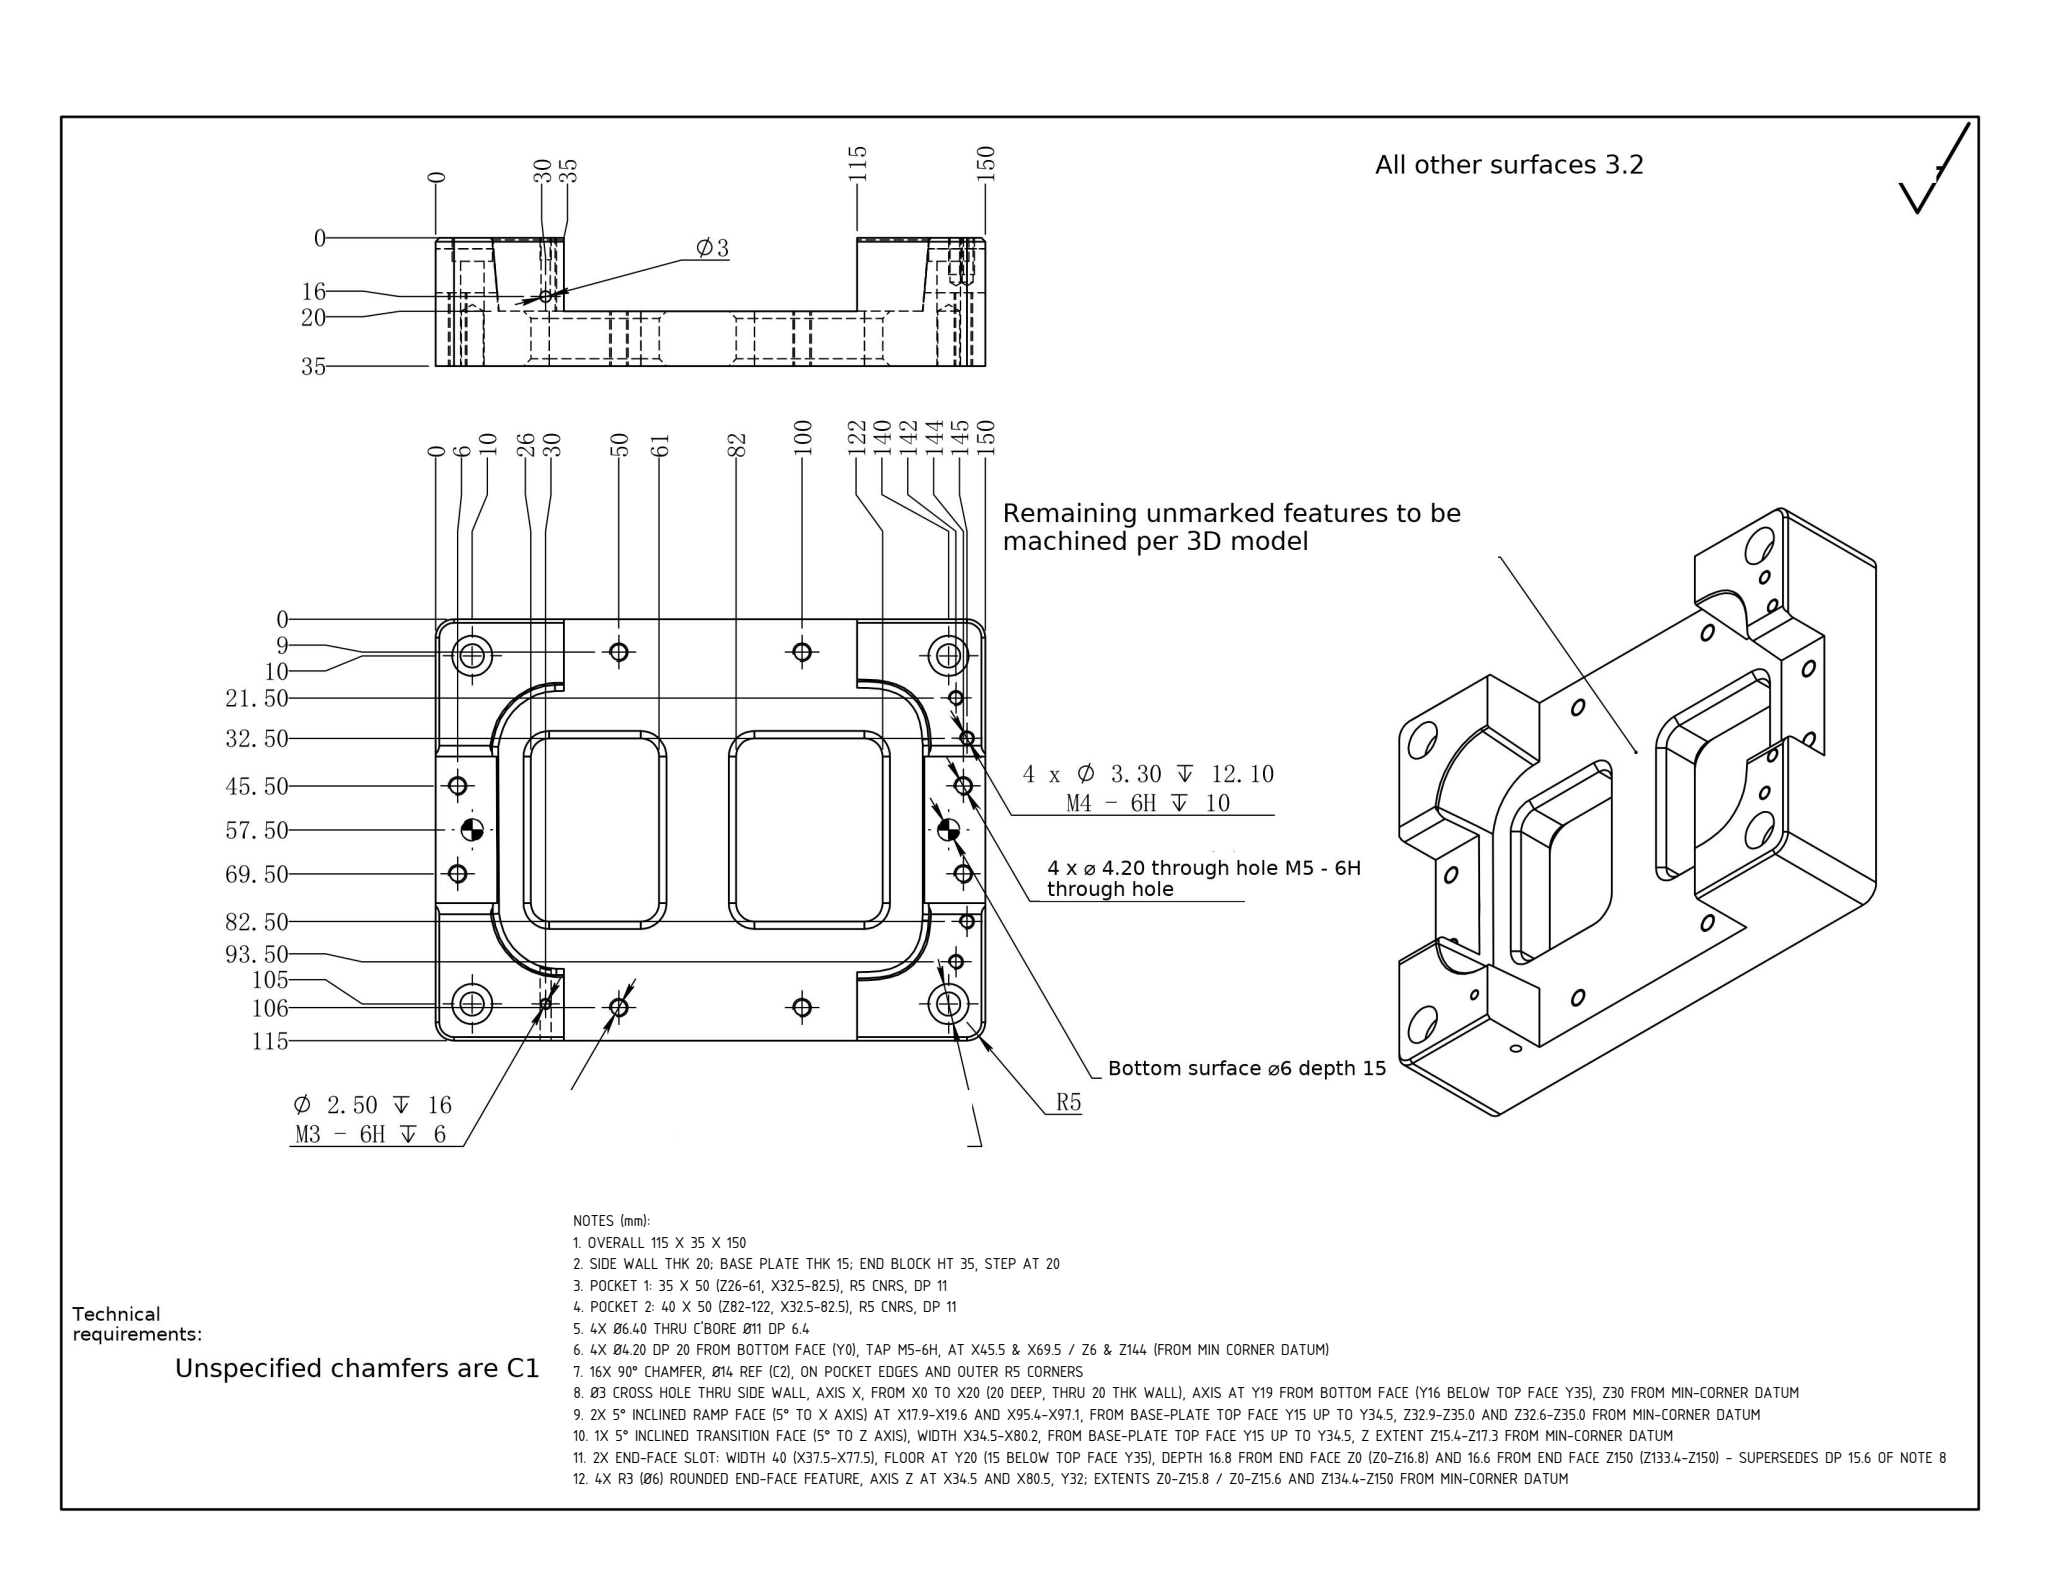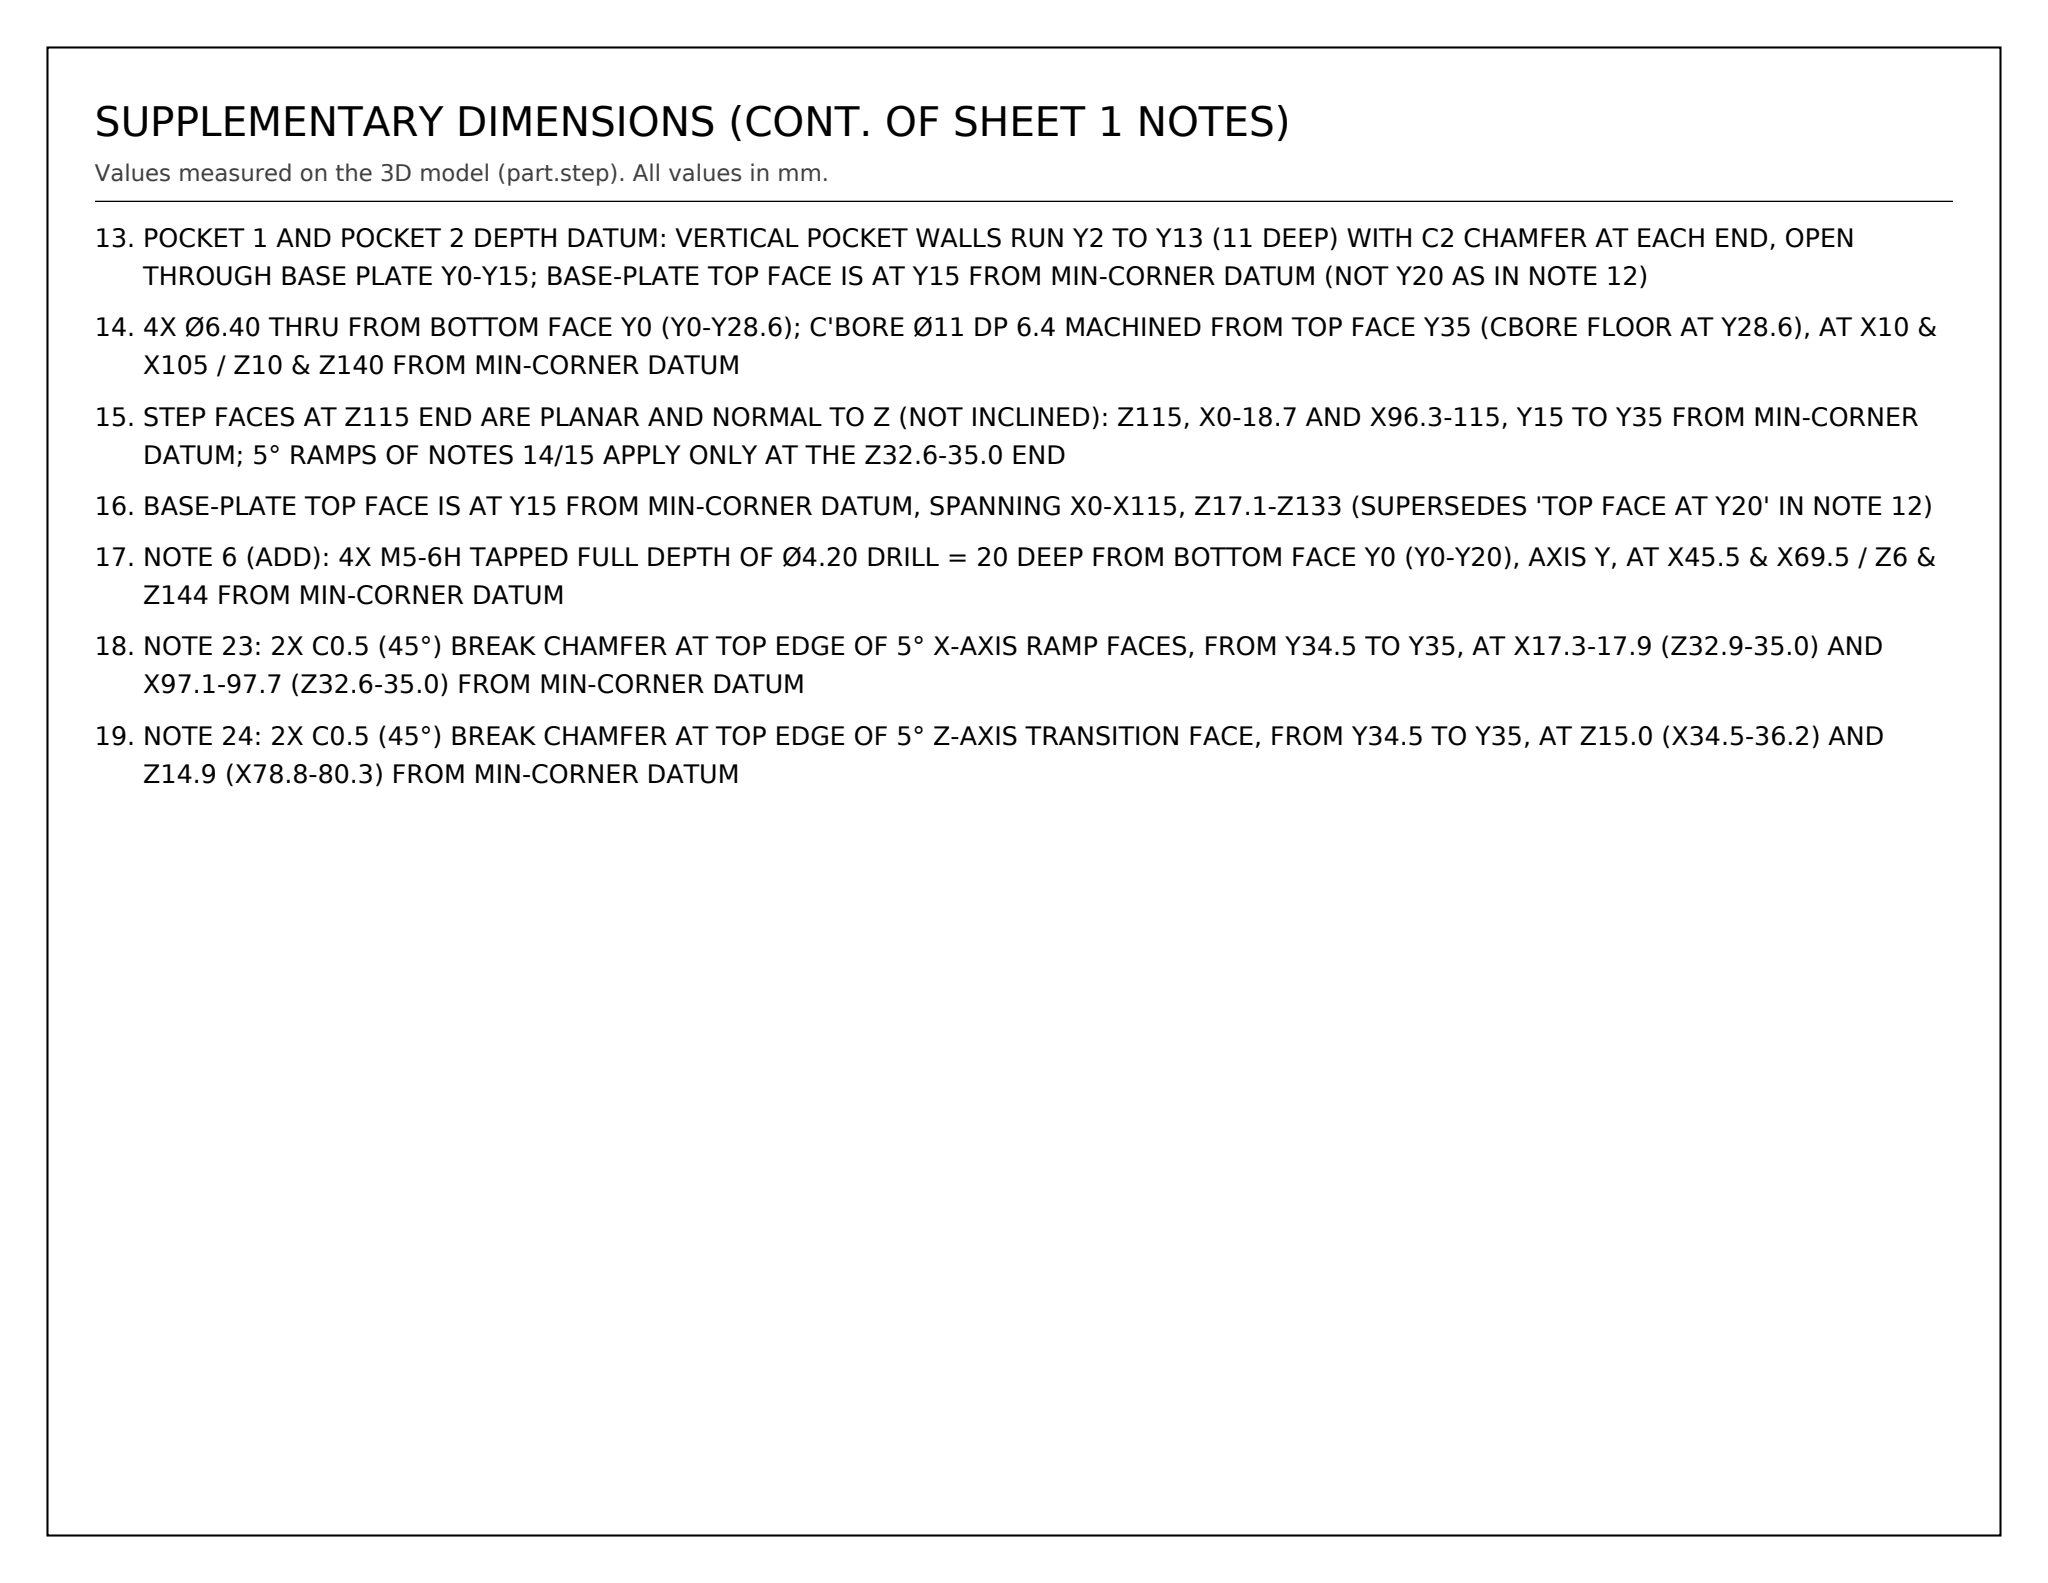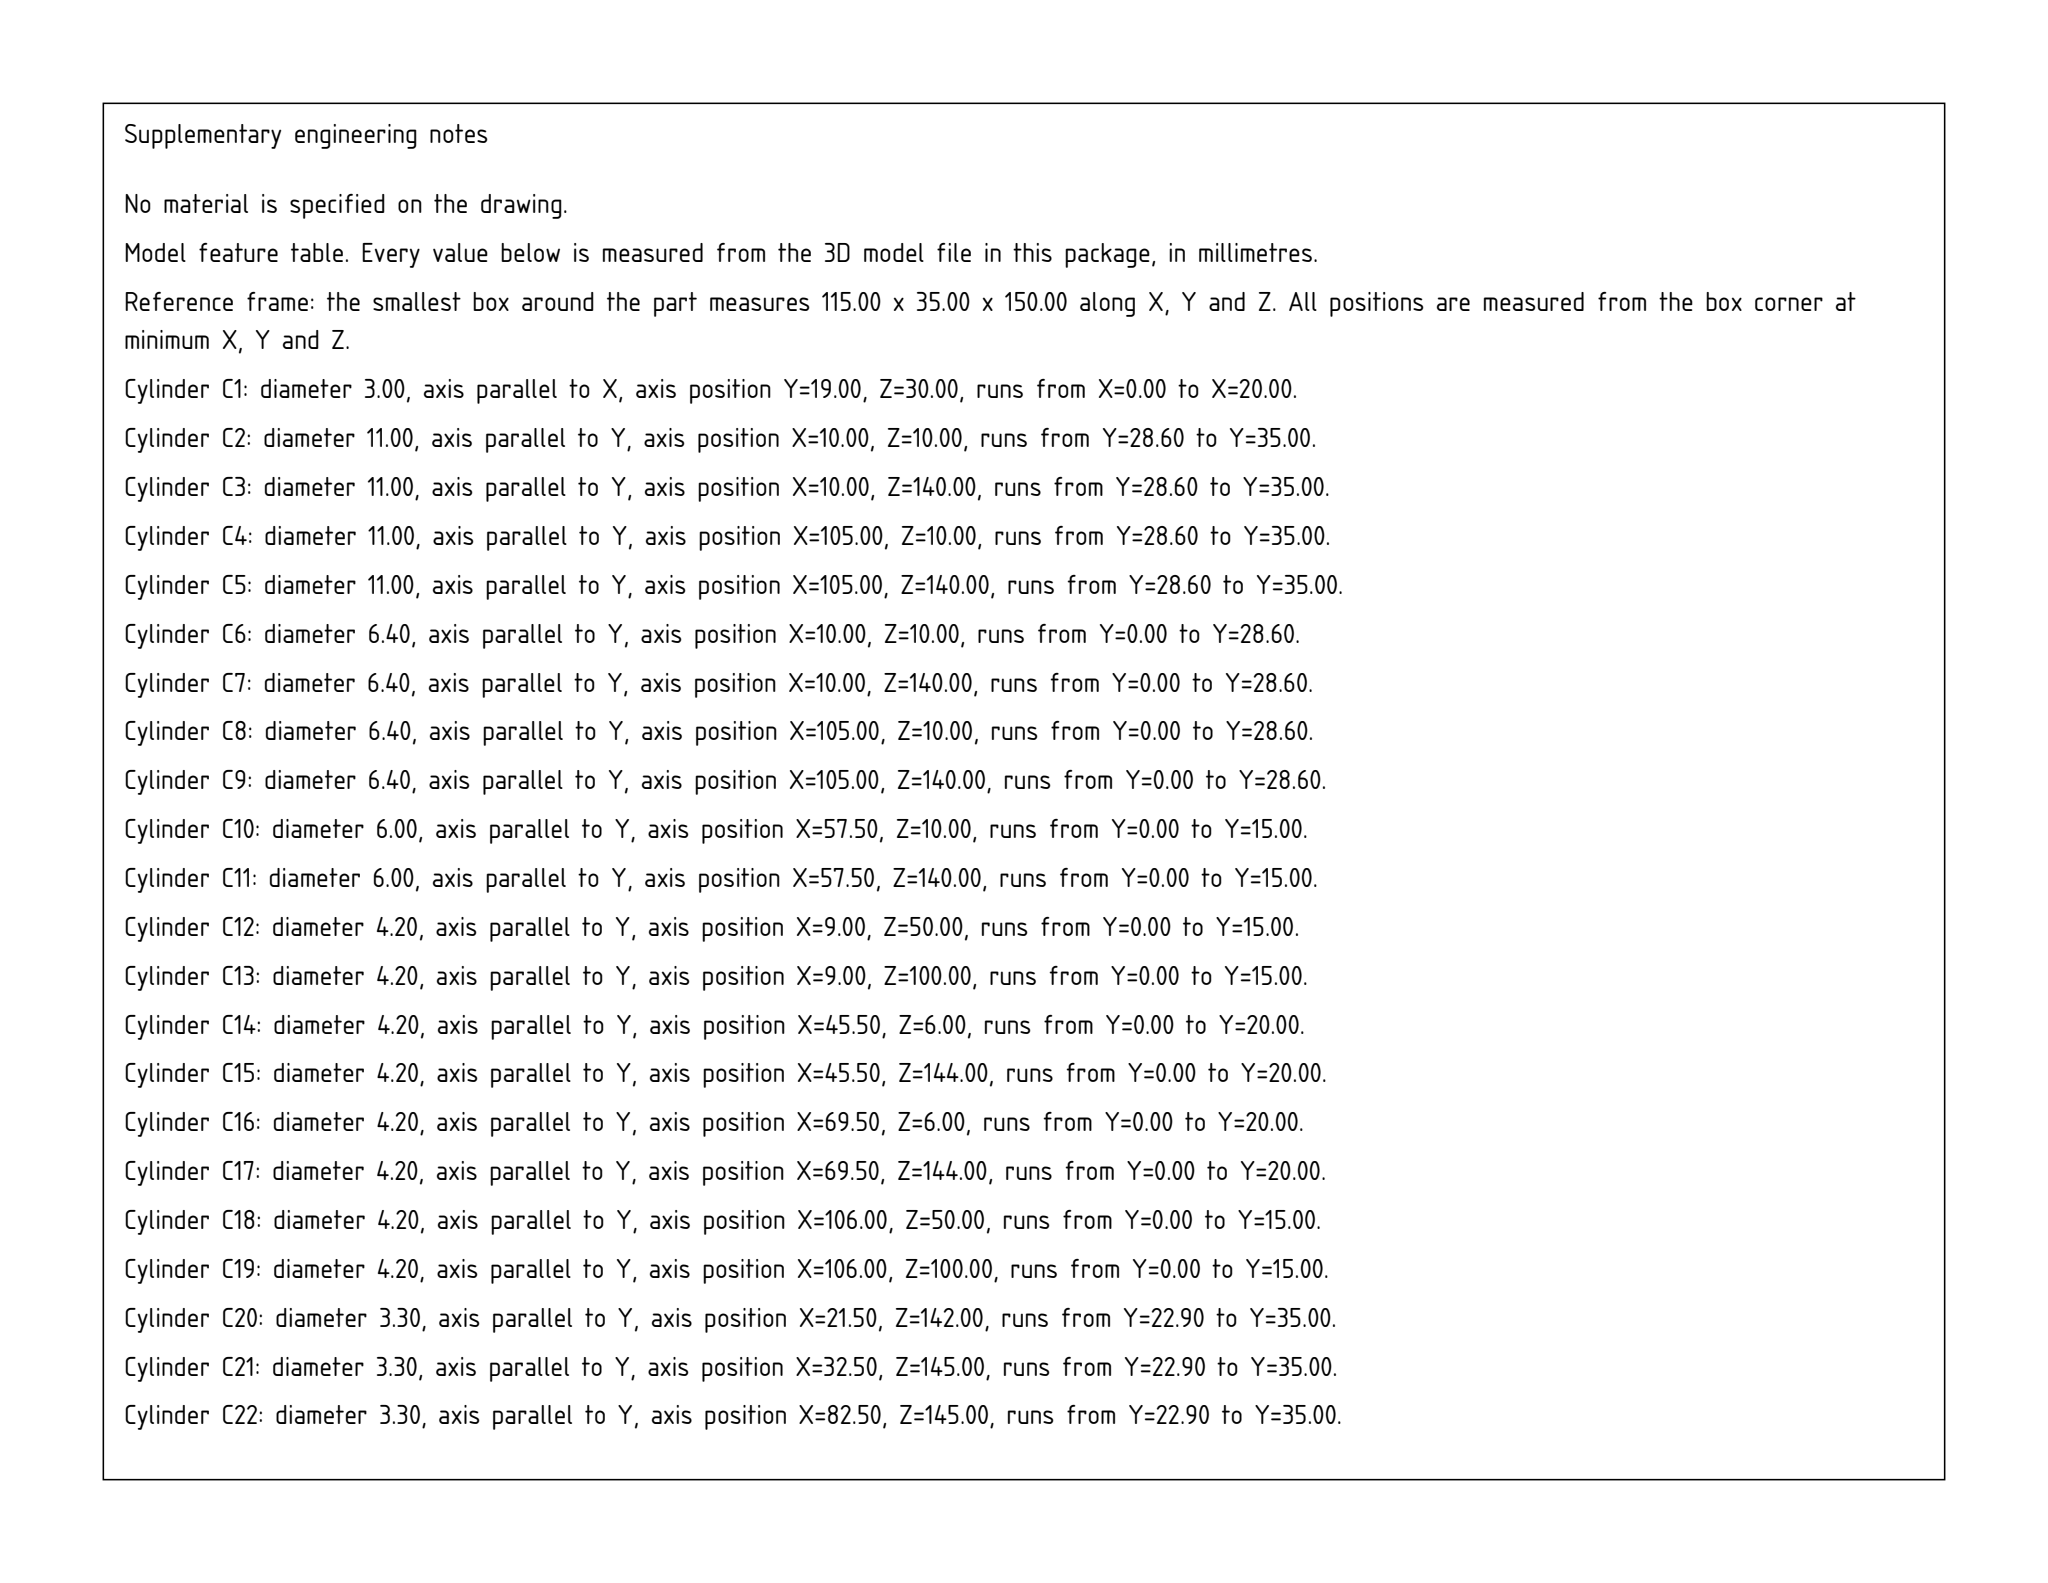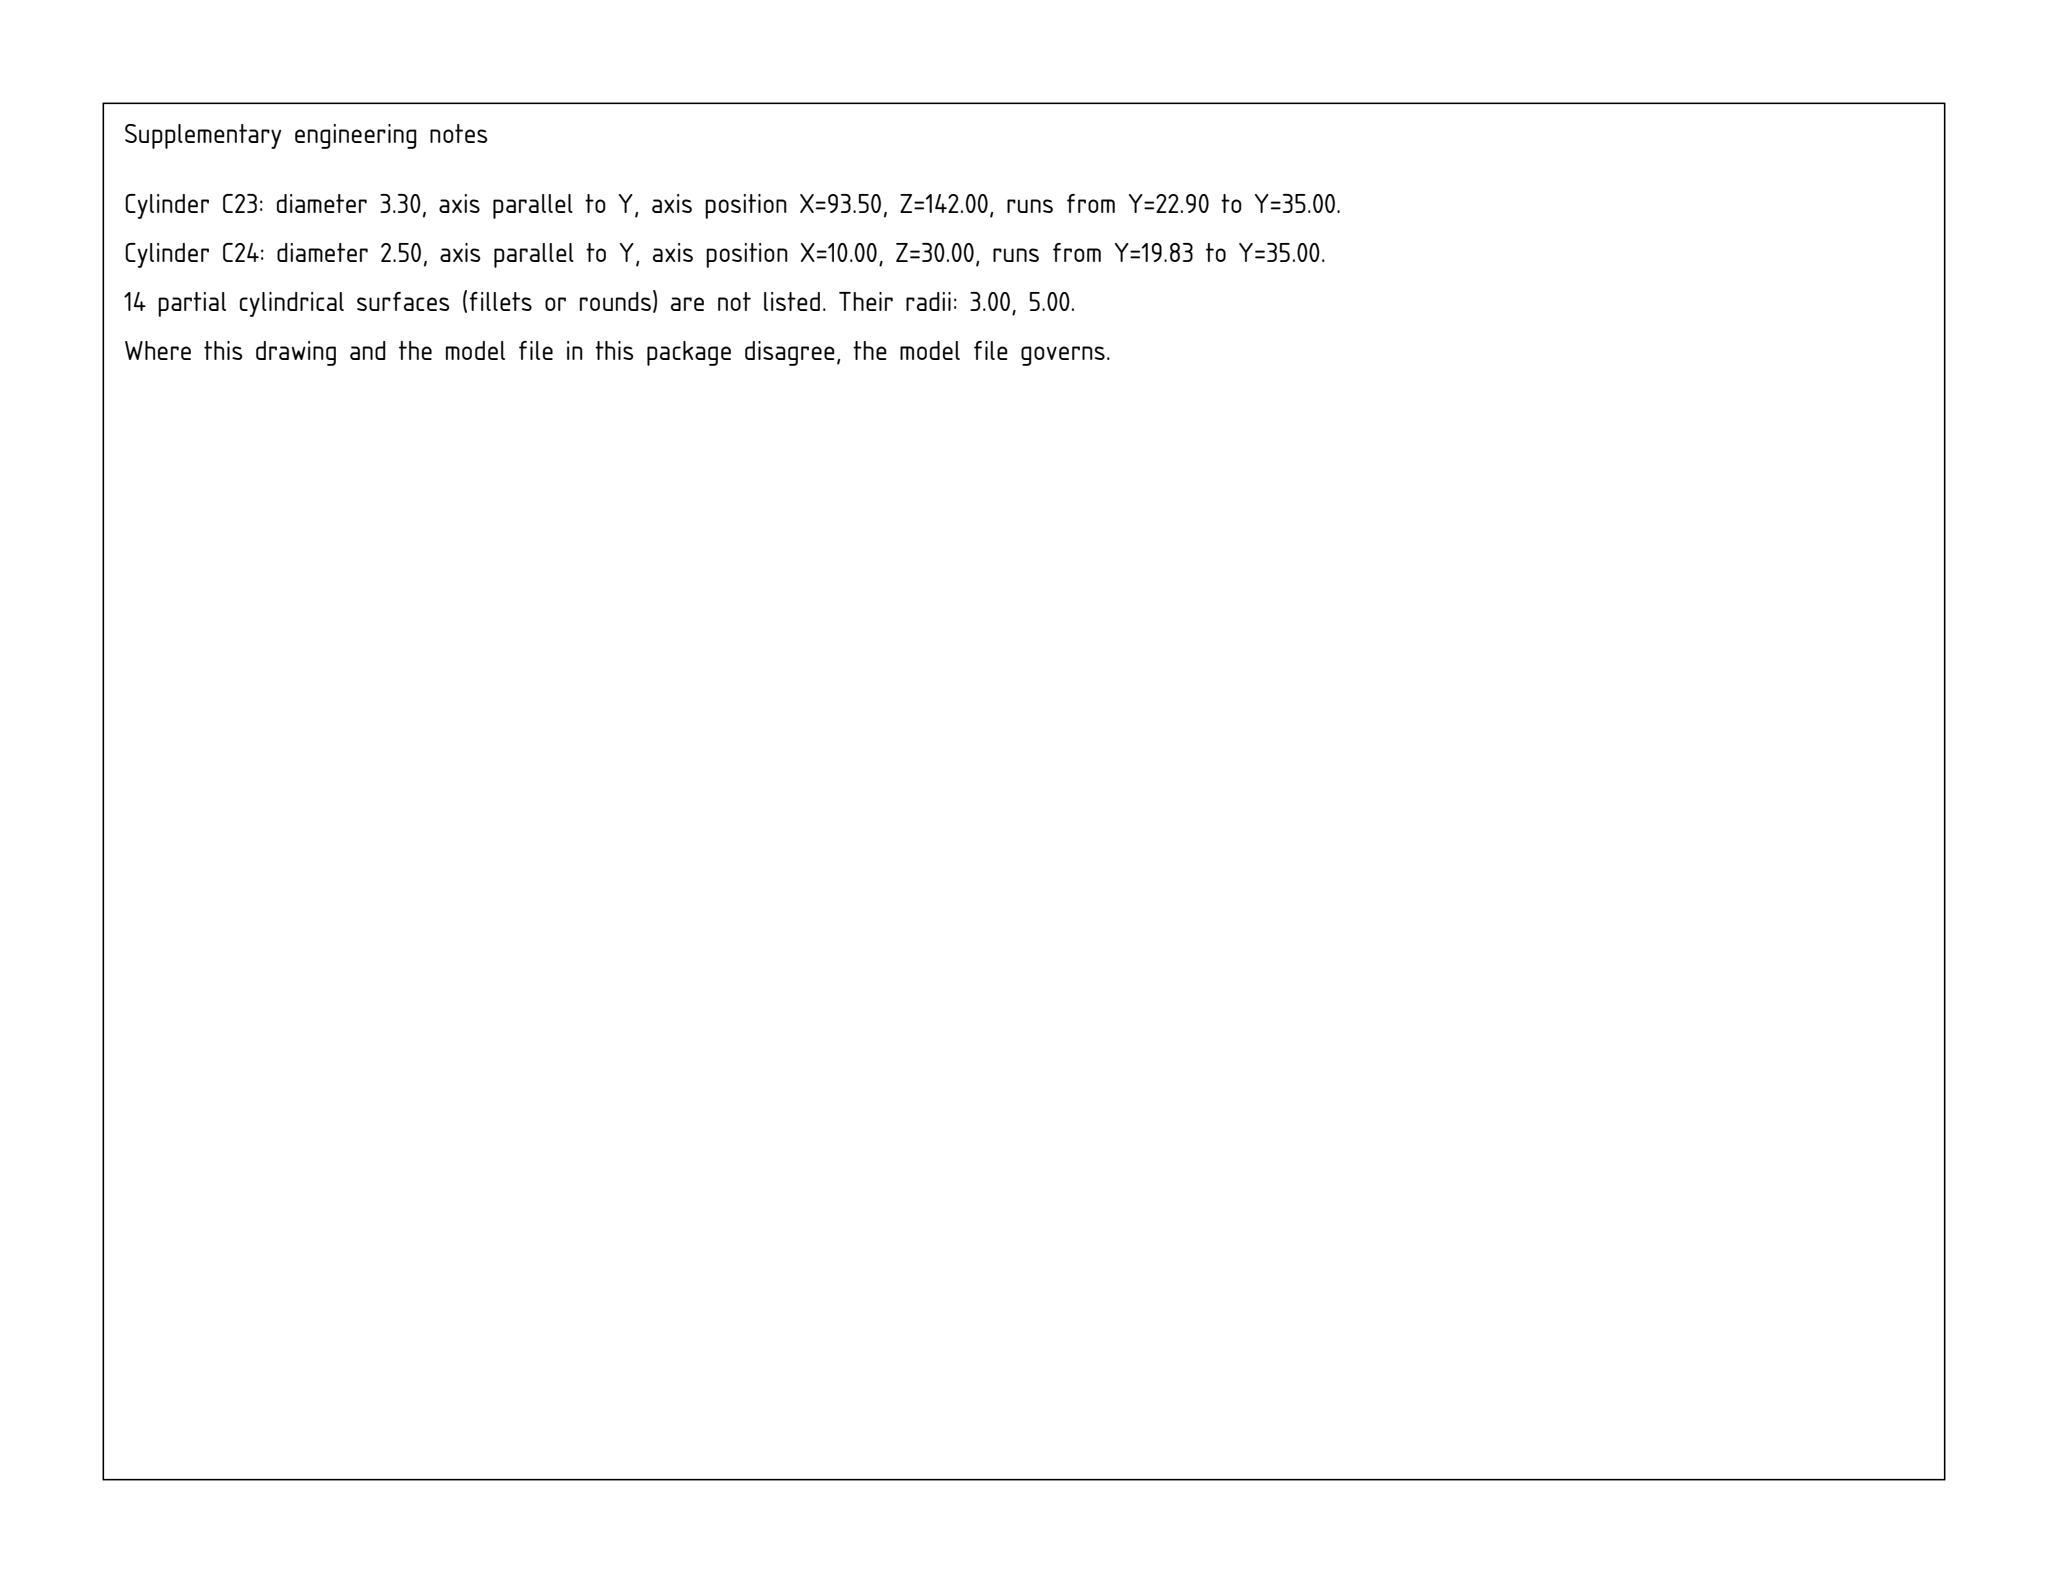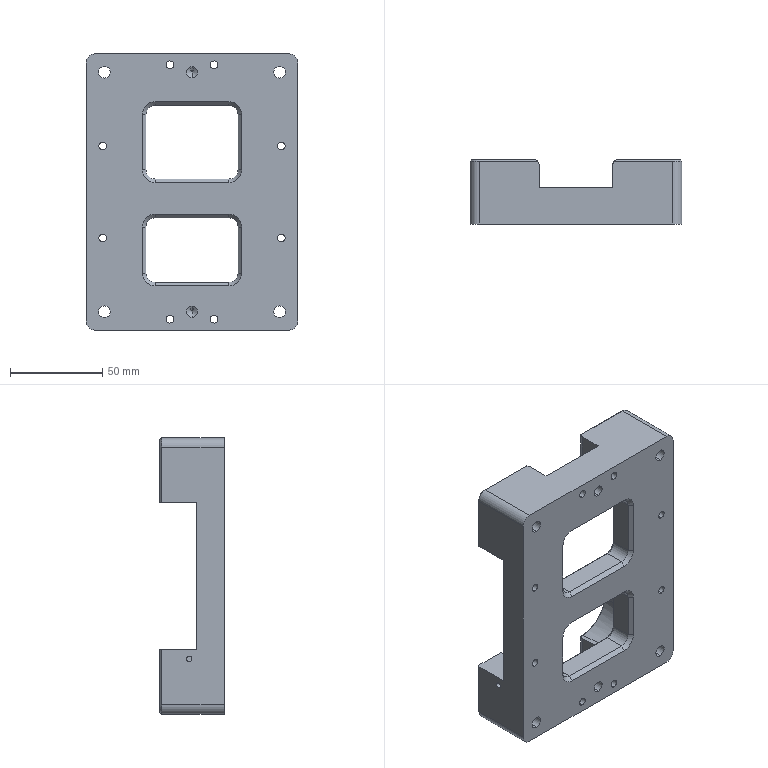Part | SolidWorks | mm | 1 solid | 173 faces | box 115 x 35 x 150 mm | volume 278458 mm3 | plane 65 | cylinder 64 | cone 32 | spline 12 | commonest cylinder face diameters 4.2 x16 10 x12 3.3 x8 6.4 x8 6 x8 11 x8 2.5 x2 3 x2
Drawing notes:
OVERALL 115 X 35 X 150 | from the solid: bbox_xyz 115.001 x 35.001 x 150.001
SIDE WALL THK 20; BASE PLATE THK 15; END BLOCK HT 35, STEP AT 20 | from the solid: x planes 0 & 20; y planes 0,15,20,35 (bbox y=35)
POCKET 1: 35 X 50 (Z26-61, X32.5-82.5), R5 CNRS, DP 11 | from the solid: D10 y-axis cnr cyls x37.5/77.5, z31/56, len 11; planes z26,z61,x32.5,x82.5
POCKET 2: 40 X 50 (Z82-122, X32.5-82.5), R5 CNRS, DP 11 | from the solid: D10 y-axis cnr cyls x37.5/77.5, z87/117, len 11; planes z82,z122
4X Ø6.40 THRU C'BORE Ø11 DP 6.4 | from the solid: D11 y cyls len 6.4 at (10,10),(10,140),(105,10),(105,140) over D6.4 len 28.6
4X Ø4.20 DP 20 FROM BOTTOM FACE (Y0), TAP M5-6H, AT X45.5 & X69.5 / Z6 & Z144 (FROM MIN CORNER DATUM) | from the solid: hole/bore 4.2 axis y at (45.5,6), (45.5,144), (69.5,6), (69.5,144) each 'from 0 to 20' in y, i.e. open at bottom face Y0, depth 20 (not from top face Y35)
16X 90° CHAMFER, Ø14 REF (C2), ON POCKET EDGES AND OUTER R5 CORNERS | from the solid: cones [90.0, 14.0, 16]
Ø3 CROSS HOLE THRU SIDE WALL, AXIS X, FROM X0 TO X20 (20 DEEP, THRU 20 THK WALL), AXIS AT Y19 FROM BOTTOM FACE (Y16 BELOW TOP FACE Y35), Z30 FROM MIN-CORNER DATUM | from the solid: cylinders: hole/bore dia 3.0, axis x, axis_pos [y=19.0, z=30.0], from 0.0 to 20.0, 360 deg
2X 5° INCLINED RAMP FACE (5° TO X AXIS) AT X17.9-X19.6 AND X95.4-X97.1, FROM BASE-PLATE TOP FACE Y15 UP TO Y34.5, Z32.9-Z35.0 AND Z32.6-Z35.0 FROM MIN-CORNER DATUM | from the solid: inclined_planes: angle_to_xyz_axes [5.0,85.0,89.4] bbox_from [17.9,15.0,32.9] size [1.7,19.5,2.1]; and bbox_from [95.4,15.0,32.6] size [1.7,19.5,2.4]
1X 5° INCLINED TRANSITION FACE (5° TO Z AXIS), WIDTH X34.5-X80.2, FROM BASE-PLATE TOP FACE Y15 UP TO Y34.5, Z EXTENT Z15.4-Z17.3 FROM MIN-CORNER DATUM | from the solid: inclined_planes: angle_to_xyz_axes [89.8,85.0,5.0] bbox_from [34.5,15.0,15.4] size [45.7,19.5,1.9]
2X END-FACE SLOT: WIDTH 40 (X37.5-X77.5), FLOOR AT Y20 (15 BELOW TOP FACE Y35), DEPTH 16.8 FROM END FACE Z0 (Z0-Z16.8) AND 16.6 FROM END FACE Z150 (Z133.4-Z150) - SUPERSEDES DP 15.6 OF NOTE 8 | from the solid: axis_planes: x=37.5 extent y[20.0,32.0] z[0.0,16.8]; x=77.5 extent y[20.0,32.0] z[0.0,16.7]; y=20.0 extent x[37.5,77.5] z[0.0,16.8] and z[133.4,150.0]
4X R3 (Ø6) ROUNDED END-FACE FEATURE, AXIS Z AT X34.5 AND X80.5, Y32; EXTENTS Z0-Z15.8 / Z0-Z15.6 AND Z134.4-Z150 FROM MIN-CORNER DATUM | from the solid: cylinders: convex arc dia 6.0 axis z at [34.5,32.0] from 0.0 to 15.8 and from 134.4 to 150.0; at [80.5,32.0] from 0.0 to 15.6 and from 134.4 to 150.0
POCKET 1 AND POCKET 2 DEPTH DATUM: VERTICAL POCKET WALLS RUN Y2 TO Y13 (11 DEEP) WITH C2 CHAMFER AT EACH END, OPEN THROUGH BASE PLATE Y0-Y15; BASE-PLATE TOP FACE IS AT Y15 FROM MIN-CORNER DATUM (NOT Y20 AS IN NOTE 12) | from the solid: cylinders: pocket corner arcs dia 10 axis y from 2.0 to 13.0; axis_planes y=15.0 extent x[0.0,115.0] z[17.1,133.0] area 7294; inclined_planes 45° chamfers bbox_from [30.5,0.0,31.0] and [30.5,13.0,31.0] size [2,2,25]
4X Ø6.40 THRU FROM BOTTOM FACE Y0 (Y0-Y28.6); C'BORE Ø11 DP 6.4 MACHINED FROM TOP FACE Y35 (CBORE FLOOR AT Y28.6), AT X10 & X105 / Z10 & Z140 FROM MIN-CORNER DATUM | from the solid: cylinders: dia 6.4 axis y from 0.0 to 28.6 and dia 11.0 axis y from 28.6 to 35.0 at [10/105, -, 10/140]; axis_plane y=28.6 extents x4.5-15.5 / 99.5-110.5
STEP FACES AT Z115 END ARE PLANAR AND NORMAL TO Z (NOT INCLINED): Z115, X0-18.7 AND X96.3-115, Y15 TO Y35 FROM MIN-CORNER DATUM; 5° RAMPS OF NOTES 14/15 APPLY ONLY AT THE Z32.6-35.0 END | from the solid: axis_planes: z=115, extents {x:[0,18.7], y:[15,35]} and {x:[96.3,115], y:[15,35]}; inclined 5° planes exist only at bbox_from x17.9/x95.4, z32.9/z32.6
BASE-PLATE TOP FACE IS AT Y15 FROM MIN-CORNER DATUM, SPANNING X0-X115, Z17.1-Z133 (SUPERSEDES 'TOP FACE AT Y20' IN NOTE 12) | from the solid: axis_plane y=15.0 extent {x:[0,115], z:[17.1,133.0]}, area 7294
NOTE 6 (ADD): 4X M5-6H TAPPED FULL DEPTH OF Ø4.20 DRILL = 20 DEEP FROM BOTTOM FACE Y0 (Y0-Y20), AXIS Y, AT X45.5 & X69.5 / Z6 & Z144 FROM MIN-CORNER DATUM | from the solid: cylinders: hole/bore Ø4.2 axis y at (45.5,-,6), (45.5,-,144), (69.5,-,6), (69.5,-,144), from 0.0 to 20.0
NOTE 23: 2X C0.5 (45°) BREAK CHAMFER AT TOP EDGE OF 5° X-AXIS RAMP FACES, FROM Y34.5 TO Y35, AT X17.3-17.9 (Z32.9-35.0) AND X97.1-97.7 (Z32.6-35.0) FROM MIN-CORNER DATUM | from the solid: inclined_planes: angle_to_xyz_axes [45,45,89.5] bbox_from [17.3,34.5,32.9] size [0.6,0.5,2.1] and bbox_from [97.1,34.5,32.6] size [0.6,0.5,2.4]
NOTE 24: 2X C0.5 (45°) BREAK CHAMFER AT TOP EDGE OF 5° Z-AXIS TRANSITION FACE, FROM Y34.5 TO Y35, AT Z15.0 (X34.5-36.2) AND Z14.9 (X78.8-80.3) FROM MIN-CORNER DATUM | from the solid: inclined_planes: angle_to_xyz_axes [89.8,45,45] bbox_from [34.5,34.5,15.0] size [1.7,0.5,0.6] and bbox_from [78.8,34.5,14.9] size [1.5,0.5,0.5]